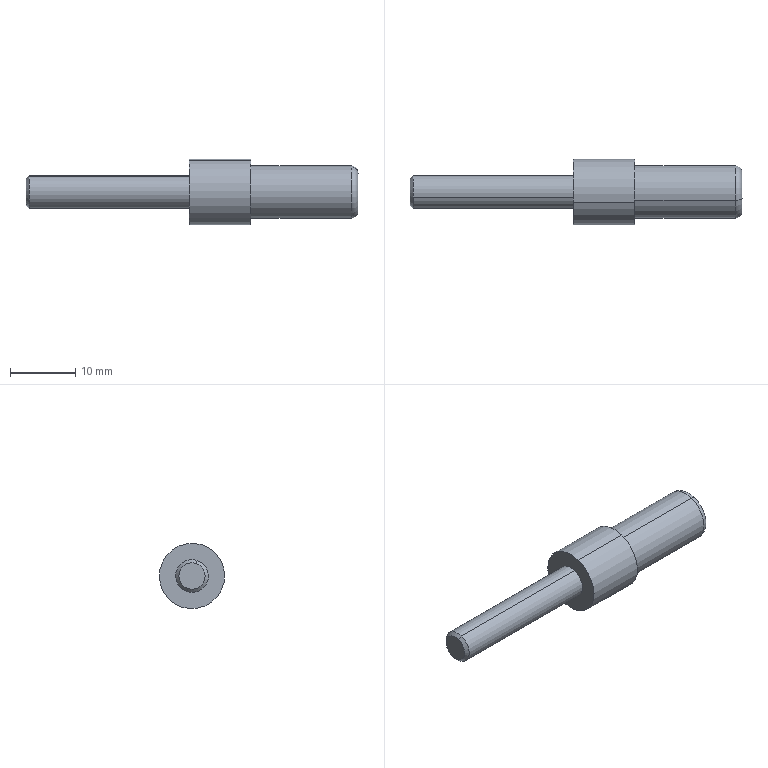Component | SolidWorks | SL010-LeftStreamline-1-1_SL010-2M-0112-000-2-1-1_SL010-CLDM5_25_B-1-1_SL010-_CLDM5_25_B_1_2-1-1 | 1 solid | 21 faces | box 50.8 x 10 x 10 mm | volume 2023 mm3 | plane 11 | cylinder 6 | torus 2 | cone 2 | commonest cylinder face diameters 8 x2 10 x2 5 x2
STEP:
#1=COLOUR_RGB('',0.7922,0.8196,0.9333);
#2=FILL_AREA_STYLE_COLOUR('',#1);
#3=FILL_AREA_STYLE('',(#2));
#4=SURFACE_STYLE_FILL_AREA(#3);
#5=SURFACE_SIDE_STYLE('',(#4));
#6=SURFACE_STYLE_USAGE(.BOTH.,#5);
#7=PRESENTATION_STYLE_ASSIGNMENT((#6));
#8=CARTESIAN_POINT('',(-5.283,-6.018,-28.334));
#9=VERTEX_POINT('',#8);
#10=CARTESIAN_POINT('',(-5.283,-5.973,-28.283));
#11=VERTEX_POINT('',#10);
#12=CARTESIAN_POINT('',(-5.283,-5.995,-28.308));
#13=DIRECTION('',(0.,0.665,0.7469));
#14=VECTOR('',#13,39.37);
#15=LINE('',#12,#14);
#16=EDGE_CURVE('',#9,#11,#15,.T.);
#17=ORIENTED_EDGE('',*,*,#16,.T.);
#18=CARTESIAN_POINT('',(-5.402,-5.973,-28.283));
#19=VERTEX_POINT('',#18);
#20=CARTESIAN_POINT('',(-5.165,-5.973,-28.283));
#21=DIRECTION('',(-1.,-0.,0.));
#22=VECTOR('',#21,39.37);
#23=LINE('',#20,#22);
#24=EDGE_CURVE('',#11,#19,#23,.T.);
#25=ORIENTED_EDGE('',*,*,#24,.T.);
#26=CARTESIAN_POINT('',(-5.402,-6.018,-28.334));
#27=VERTEX_POINT('',#26);
#28=CARTESIAN_POINT('',(-5.402,-6.018,-28.334));
#29=DIRECTION('',(0.,0.665,0.7469));
#30=VECTOR('',#29,39.37);
#31=LINE('',#28,#30);
#32=EDGE_CURVE('',#27,#19,#31,.T.);
#33=ORIENTED_EDGE('',*,*,#32,.F.);
#34=CARTESIAN_POINT('',(-5.165,-6.018,-28.334));
#35=DIRECTION('',(-1.,-0.,0.));
#36=VECTOR('',#35,39.37);
#37=LINE('',#34,#36);
#38=EDGE_CURVE('',#9,#27,#37,.T.);
#39=ORIENTED_EDGE('',*,*,#38,.F.);
#40=EDGE_LOOP('',(#17,#25,#33,#39));
#41=FACE_OUTER_BOUND('',#40,.T.);
#42=CARTESIAN_POINT('',(-5.165,-6.018,-28.334));
#43=DIRECTION('',(0.,-0.7469,0.665));
#44=DIRECTION('',(-0.,-0.665,-0.7469));
#45=AXIS2_PLACEMENT_3D('',#42,#43,#44);
#46=PLANE('',#45);
#47=ADVANCED_FACE('',(#41),#46,.T.);
#48=CARTESIAN_POINT('',(-5.283,-6.085,-28.32));
#49=VERTEX_POINT('',#48);
#50=CARTESIAN_POINT('',(-5.283,-6.051,-28.327));
#51=DIRECTION('',(-0.,0.9793,-0.2025));
#52=VECTOR('',#51,39.37);
#53=LINE('',#50,#52);
#54=EDGE_CURVE('',#49,#9,#53,.T.);
#55=ORIENTED_EDGE('',*,*,#54,.T.);
#56=ORIENTED_EDGE('',*,*,#38,.T.);
#57=CARTESIAN_POINT('',(-5.402,-6.085,-28.32));
#58=VERTEX_POINT('',#57);
#59=CARTESIAN_POINT('',(-5.402,-6.085,-28.32));
#60=DIRECTION('',(-0.,0.9793,-0.2025));
#61=VECTOR('',#60,39.37);
#62=LINE('',#59,#61);
#63=EDGE_CURVE('',#58,#27,#62,.T.);
#64=ORIENTED_EDGE('',*,*,#63,.F.);
#65=CARTESIAN_POINT('',(-5.165,-6.085,-28.32));
#66=DIRECTION('',(-1.,-0.,0.));
#67=VECTOR('',#66,39.37);
#68=LINE('',#65,#67);
#69=EDGE_CURVE('',#49,#58,#68,.T.);
#70=ORIENTED_EDGE('',*,*,#69,.F.);
#71=EDGE_LOOP('',(#55,#56,#64,#70));
#72=FACE_OUTER_BOUND('',#71,.T.);
#73=CARTESIAN_POINT('',(-5.165,-6.085,-28.32));
#74=DIRECTION('',(0.,0.2025,0.9793));
#75=DIRECTION('',(0.,-0.9793,0.2025));
#76=AXIS2_PLACEMENT_3D('',#73,#74,#75);
#77=PLANE('',#76);
#78=ADVANCED_FACE('',(#72),#77,.T.);
#79=CARTESIAN_POINT('',(-5.283,-6.106,-28.255));
#80=VERTEX_POINT('',#79);
#81=CARTESIAN_POINT('',(-5.402,-6.106,-28.255));
#82=VERTEX_POINT('',#81);
#83=CARTESIAN_POINT('',(-5.165,-6.106,-28.255));
#84=DIRECTION('',(-1.,-0.,0.));
#85=VECTOR('',#84,39.37);
#86=LINE('',#83,#85);
#87=EDGE_CURVE('',#80,#82,#86,.T.);
#88=ORIENTED_EDGE('',*,*,#87,.F.);
#89=CARTESIAN_POINT('',(-5.283,-6.096,-28.288));
#90=DIRECTION('',(-0.,0.3143,-0.9493));
#91=VECTOR('',#90,39.37);
#92=LINE('',#89,#91);
#93=EDGE_CURVE('',#80,#49,#92,.T.);
#94=ORIENTED_EDGE('',*,*,#93,.T.);
#95=ORIENTED_EDGE('',*,*,#69,.T.);
#96=CARTESIAN_POINT('',(-5.402,-6.106,-28.255));
#97=DIRECTION('',(-0.,0.3143,-0.9493));
#98=VECTOR('',#97,39.37);
#99=LINE('',#96,#98);
#100=EDGE_CURVE('',#82,#58,#99,.T.);
#101=ORIENTED_EDGE('',*,*,#100,.F.);
#102=EDGE_LOOP('',(#88,#94,#95,#101));
#103=FACE_OUTER_BOUND('',#102,.T.);
#104=CARTESIAN_POINT('',(-5.165,-6.106,-28.255));
#105=DIRECTION('',(0.,0.9493,0.3143));
#106=DIRECTION('',(0.,-0.3143,0.9493));
#107=AXIS2_PLACEMENT_3D('',#104,#105,#106);
#108=PLANE('',#107);
#109=ADVANCED_FACE('',(#103),#108,.T.);
#110=CARTESIAN_POINT('',(-5.402,-5.994,-28.218));
#111=VERTEX_POINT('',#110);
#112=CARTESIAN_POINT('',(-5.402,-5.973,-28.283));
#113=DIRECTION('',(0.,-0.3143,0.9493));
#114=VECTOR('',#113,39.37);
#115=LINE('',#112,#114);
#116=EDGE_CURVE('',#19,#111,#115,.T.);
#117=ORIENTED_EDGE('',*,*,#116,.T.);
#118=CARTESIAN_POINT('',(-5.402,-6.061,-28.204));
#119=VERTEX_POINT('',#118);
#120=CARTESIAN_POINT('',(-5.402,-5.994,-28.218));
#121=DIRECTION('',(0.,-0.9793,0.2025));
#122=VECTOR('',#121,39.37);
#123=LINE('',#120,#122);
#124=EDGE_CURVE('',#111,#119,#123,.T.);
#125=ORIENTED_EDGE('',*,*,#124,.T.);
#126=CARTESIAN_POINT('',(-5.402,-6.061,-28.204));
#127=DIRECTION('',(-0.,-0.665,-0.7469));
#128=VECTOR('',#127,39.37);
#129=LINE('',#126,#128);
#130=EDGE_CURVE('',#119,#82,#129,.T.);
#131=ORIENTED_EDGE('',*,*,#130,.T.);
#132=ORIENTED_EDGE('',*,*,#100,.T.);
#133=ORIENTED_EDGE('',*,*,#63,.T.);
#134=ORIENTED_EDGE('',*,*,#32,.T.);
#135=EDGE_LOOP('',(#117,#125,#131,#132,#133,#134));
#136=FACE_OUTER_BOUND('',#135,.T.);
#137=CARTESIAN_POINT('',(-5.402,-6.04,-28.269));
#138=DIRECTION('',(1.,0.,-0.));
#139=DIRECTION('',(0.,-0.3143,0.9493));
#140=AXIS2_PLACEMENT_3D('',#137,#138,#139);
#141=PLANE('',#140);
#142=ADVANCED_FACE('',(#136),#141,.T.);
#143=CARTESIAN_POINT('',(-5.283,-6.061,-28.204));
#144=VERTEX_POINT('',#143);
#145=CARTESIAN_POINT('',(-5.283,-6.084,-28.23));
#146=DIRECTION('',(-0.,-0.665,-0.7469));
#147=VECTOR('',#146,39.37);
#148=LINE('',#145,#147);
#149=EDGE_CURVE('',#144,#80,#148,.T.);
#150=ORIENTED_EDGE('',*,*,#149,.T.);
#151=ORIENTED_EDGE('',*,*,#87,.T.);
#152=ORIENTED_EDGE('',*,*,#130,.F.);
#153=CARTESIAN_POINT('',(-5.165,-6.061,-28.204));
#154=DIRECTION('',(-1.,-0.,0.));
#155=VECTOR('',#154,39.37);
#156=LINE('',#153,#155);
#157=EDGE_CURVE('',#144,#119,#156,.T.);
#158=ORIENTED_EDGE('',*,*,#157,.F.);
#159=EDGE_LOOP('',(#150,#151,#152,#158));
#160=FACE_OUTER_BOUND('',#159,.T.);
#161=CARTESIAN_POINT('',(-5.165,-6.061,-28.204));
#162=DIRECTION('',(-0.,0.7469,-0.665));
#163=DIRECTION('',(0.,0.665,0.7469));
#164=AXIS2_PLACEMENT_3D('',#161,#162,#163);
#165=PLANE('',#164);
#166=ADVANCED_FACE('',(#160),#165,.T.);
#167=CARTESIAN_POINT('',(-5.283,-5.994,-28.218));
#168=VERTEX_POINT('',#167);
#169=CARTESIAN_POINT('',(-5.283,-6.028,-28.211));
#170=DIRECTION('',(0.,-0.9793,0.2025));
#171=VECTOR('',#170,39.37);
#172=LINE('',#169,#171);
#173=EDGE_CURVE('',#168,#144,#172,.T.);
#174=ORIENTED_EDGE('',*,*,#173,.T.);
#175=ORIENTED_EDGE('',*,*,#157,.T.);
#176=ORIENTED_EDGE('',*,*,#124,.F.);
#177=CARTESIAN_POINT('',(-5.165,-5.994,-28.218));
#178=DIRECTION('',(-1.,-0.,0.));
#179=VECTOR('',#178,39.37);
#180=LINE('',#177,#179);
#181=EDGE_CURVE('',#168,#111,#180,.T.);
#182=ORIENTED_EDGE('',*,*,#181,.F.);
#183=EDGE_LOOP('',(#174,#175,#176,#182));
#184=FACE_OUTER_BOUND('',#183,.T.);
#185=CARTESIAN_POINT('',(-5.165,-5.994,-28.218));
#186=DIRECTION('',(-0.,-0.2025,-0.9793));
#187=DIRECTION('',(-0.,0.9793,-0.2025));
#188=AXIS2_PLACEMENT_3D('',#185,#186,#187);
#189=PLANE('',#188);
#190=ADVANCED_FACE('',(#184),#189,.T.);
#191=CARTESIAN_POINT('',(-5.283,-5.983,-28.251));
#192=DIRECTION('',(0.,-0.3143,0.9493));
#193=VECTOR('',#192,39.37);
#194=LINE('',#191,#193);
#195=EDGE_CURVE('',#11,#168,#194,.T.);
#196=ORIENTED_EDGE('',*,*,#195,.T.);
#197=ORIENTED_EDGE('',*,*,#181,.T.);
#198=ORIENTED_EDGE('',*,*,#116,.F.);
#199=ORIENTED_EDGE('',*,*,#24,.F.);
#200=EDGE_LOOP('',(#196,#197,#198,#199));
#201=FACE_OUTER_BOUND('',#200,.T.);
#202=CARTESIAN_POINT('',(-5.165,-5.973,-28.283));
#203=DIRECTION('',(0.,-0.9493,-0.3143));
#204=DIRECTION('',(-0.,0.3143,-0.9493));
#205=AXIS2_PLACEMENT_3D('',#202,#203,#204);
#206=PLANE('',#205);
#207=ADVANCED_FACE('',(#201),#206,.T.);
#208=CARTESIAN_POINT('',(-5.283,-6.002,-28.381));
#209=VERTEX_POINT('',#208);
#210=CARTESIAN_POINT('',(-5.283,-6.077,-28.157));
#211=VERTEX_POINT('',#210);
#212=CARTESIAN_POINT('',(-5.283,-6.04,-28.269));
#213=DIRECTION('',(-1.,-0.,0.));
#214=DIRECTION('',(0.,0.3143,-0.9493));
#215=AXIS2_PLACEMENT_3D('',#212,#213,#214);
#216=CIRCLE('',#215,0.1181);
#217=EDGE_CURVE('',#209,#211,#216,.T.);
#218=ORIENTED_EDGE('',*,*,#217,.F.);
#219=CARTESIAN_POINT('',(-5.283,-6.04,-28.269));
#220=DIRECTION('',(-1.,-0.,0.));
#221=DIRECTION('',(0.,0.3143,-0.9493));
#222=AXIS2_PLACEMENT_3D('',#219,#220,#221);
#223=CIRCLE('',#222,0.1181);
#224=EDGE_CURVE('',#211,#209,#223,.T.);
#225=ORIENTED_EDGE('',*,*,#224,.F.);
#226=EDGE_LOOP('',(#218,#225));
#227=FACE_OUTER_BOUND('',#226,.T.);
#228=ORIENTED_EDGE('',*,*,#195,.F.);
#229=ORIENTED_EDGE('',*,*,#16,.F.);
#230=ORIENTED_EDGE('',*,*,#54,.F.);
#231=ORIENTED_EDGE('',*,*,#93,.F.);
#232=ORIENTED_EDGE('',*,*,#149,.F.);
#233=ORIENTED_EDGE('',*,*,#173,.F.);
#234=EDGE_LOOP('',(#228,#229,#230,#231,#232,#233));
#235=FACE_BOUND('',#234,.T.);
#236=CARTESIAN_POINT('',(-5.283,-6.04,-28.269));
#237=DIRECTION('',(-1.,-0.,0.));
#238=DIRECTION('',(-0.,0.3143,-0.9493));
#239=AXIS2_PLACEMENT_3D('',#236,#237,#238);
#240=PLANE('',#239);
#241=ADVANCED_FACE('',(#227,#235),#240,.F.);
#242=ORIENTED_EDGE('',*,*,#224,.T.);
#243=CARTESIAN_POINT('',(-5.323,-5.99,-28.419));
#244=VERTEX_POINT('',#243);
#245=CARTESIAN_POINT('',(-5.283,-6.002,-28.381));
#246=CARTESIAN_POINT('',(-5.283,-5.999,-28.391));
#247=CARTESIAN_POINT('',(-5.288,-5.996,-28.401));
#248=CARTESIAN_POINT('',(-5.302,-5.991,-28.415));
#249=CARTESIAN_POINT('',(-5.313,-5.99,-28.419));
#250=CARTESIAN_POINT('',(-5.323,-5.99,-28.419));
#251=B_SPLINE_CURVE_WITH_KNOTS('',3,(#245,#246,#247,#248,#249,#250),.UNSPECIFIED.,.F.,.F.,(4,2,4),(0.,0.7854,1.571),.UNSPECIFIED.);
#252=EDGE_CURVE('',#209,#244,#251,.T.);
#253=ORIENTED_EDGE('',*,*,#252,.T.);
#254=CARTESIAN_POINT('',(-5.323,-6.089,-28.12));
#255=VERTEX_POINT('',#254);
#256=CARTESIAN_POINT('',(-5.323,-6.04,-28.269));
#257=DIRECTION('',(-1.,-0.,0.));
#258=DIRECTION('',(0.,0.3143,-0.9493));
#259=AXIS2_PLACEMENT_3D('',#256,#257,#258);
#260=CIRCLE('',#259,0.1575);
#261=EDGE_CURVE('',#255,#244,#260,.T.);
#262=ORIENTED_EDGE('',*,*,#261,.F.);
#263=CARTESIAN_POINT('',(-5.283,-6.077,-28.157));
#264=CARTESIAN_POINT('',(-5.283,-6.08,-28.147));
#265=CARTESIAN_POINT('',(-5.288,-6.083,-28.137));
#266=CARTESIAN_POINT('',(-5.302,-6.088,-28.124));
#267=CARTESIAN_POINT('',(-5.313,-6.089,-28.12));
#268=CARTESIAN_POINT('',(-5.323,-6.089,-28.12));
#269=B_SPLINE_CURVE_WITH_KNOTS('',3,(#263,#264,#265,#266,#267,#268),.UNSPECIFIED.,.F.,.F.,(4,2,4),(0.,0.7854,1.571),.UNSPECIFIED.);
#270=EDGE_CURVE('',#211,#255,#269,.T.);
#271=ORIENTED_EDGE('',*,*,#270,.F.);
#272=EDGE_LOOP('',(#242,#253,#262,#271));
#273=FACE_OUTER_BOUND('',#272,.T.);
#274=CARTESIAN_POINT('',(-5.323,-6.04,-28.269));
#275=DIRECTION('',(-1.,-0.,0.));
#276=DIRECTION('',(0.,-0.9493,-0.3143));
#277=AXIS2_PLACEMENT_3D('',#274,#275,#276);
#278=TOROIDAL_SURFACE('',#277,0.1181,0.03937);
#279=ADVANCED_FACE('',(#273),#278,.T.);
#280=CARTESIAN_POINT('',(-5.323,-6.04,-28.269));
#281=DIRECTION('',(-1.,-0.,0.));
#282=DIRECTION('',(0.,0.3143,-0.9493));
#283=AXIS2_PLACEMENT_3D('',#280,#281,#282);
#284=CIRCLE('',#283,0.1575);
#285=EDGE_CURVE('',#244,#255,#284,.T.);
#286=ORIENTED_EDGE('',*,*,#285,.F.);
#287=ORIENTED_EDGE('',*,*,#252,.F.);
#288=ORIENTED_EDGE('',*,*,#217,.T.);
#289=ORIENTED_EDGE('',*,*,#270,.T.);
#290=EDGE_LOOP('',(#286,#287,#288,#289));
#291=FACE_OUTER_BOUND('',#290,.T.);
#292=CARTESIAN_POINT('',(-5.323,-6.04,-28.269));
#293=DIRECTION('',(-1.,-0.,0.));
#294=DIRECTION('',(-0.,0.9493,0.3143));
#295=AXIS2_PLACEMENT_3D('',#292,#293,#294);
#296=TOROIDAL_SURFACE('',#295,0.1181,0.03937);
#297=ADVANCED_FACE('',(#291),#296,.T.);
#298=CARTESIAN_POINT('',(-5.929,-5.99,-28.419));
#299=VERTEX_POINT('',#298);
#300=CARTESIAN_POINT('',(-5.929,-6.089,-28.12));
#301=VERTEX_POINT('',#300);
#302=CARTESIAN_POINT('',(-5.929,-6.04,-28.269));
#303=DIRECTION('',(-1.,-0.,0.));
#304=DIRECTION('',(0.,0.3143,-0.9493));
#305=AXIS2_PLACEMENT_3D('',#302,#303,#304);
#306=CIRCLE('',#305,0.1575);
#307=EDGE_CURVE('',#299,#301,#306,.T.);
#308=ORIENTED_EDGE('',*,*,#307,.F.);
#309=CARTESIAN_POINT('',(-5.929,-5.99,-28.419));
#310=DIRECTION('',(1.,0.,-0.));
#311=VECTOR('',#310,39.37);
#312=LINE('',#309,#311);
#313=EDGE_CURVE('',#299,#244,#312,.T.);
#314=ORIENTED_EDGE('',*,*,#313,.T.);
#315=ORIENTED_EDGE('',*,*,#285,.T.);
#316=CARTESIAN_POINT('',(-5.929,-6.089,-28.12));
#317=DIRECTION('',(1.,0.,-0.));
#318=VECTOR('',#317,39.37);
#319=LINE('',#316,#318);
#320=EDGE_CURVE('',#301,#255,#319,.T.);
#321=ORIENTED_EDGE('',*,*,#320,.F.);
#322=EDGE_LOOP('',(#308,#314,#315,#321));
#323=FACE_OUTER_BOUND('',#322,.T.);
#324=CARTESIAN_POINT('',(-7.283,-6.04,-28.269));
#325=DIRECTION('',(1.,0.,-0.));
#326=DIRECTION('',(0.,0.9493,0.3143));
#327=AXIS2_PLACEMENT_3D('',#324,#325,#326);
#328=CYLINDRICAL_SURFACE('',#327,0.1575);
#329=ADVANCED_FACE('',(#323),#328,.T.);
#330=ORIENTED_EDGE('',*,*,#261,.T.);
#331=ORIENTED_EDGE('',*,*,#313,.F.);
#332=CARTESIAN_POINT('',(-5.929,-6.04,-28.269));
#333=DIRECTION('',(-1.,-0.,0.));
#334=DIRECTION('',(0.,0.3143,-0.9493));
#335=AXIS2_PLACEMENT_3D('',#332,#333,#334);
#336=CIRCLE('',#335,0.1575);
#337=EDGE_CURVE('',#301,#299,#336,.T.);
#338=ORIENTED_EDGE('',*,*,#337,.F.);
#339=ORIENTED_EDGE('',*,*,#320,.T.);
#340=EDGE_LOOP('',(#330,#331,#338,#339));
#341=FACE_OUTER_BOUND('',#340,.T.);
#342=CARTESIAN_POINT('',(-7.283,-6.04,-28.269));
#343=DIRECTION('',(1.,0.,-0.));
#344=DIRECTION('',(0.,-0.9493,-0.3143));
#345=AXIS2_PLACEMENT_3D('',#342,#343,#344);
#346=CYLINDRICAL_SURFACE('',#345,0.1575);
#347=ADVANCED_FACE('',(#341),#346,.T.);
#348=CARTESIAN_POINT('',(-5.929,-5.978,-28.456));
#349=VERTEX_POINT('',#348);
#350=CARTESIAN_POINT('',(-5.929,-6.101,-28.082));
#351=VERTEX_POINT('',#350);
#352=CARTESIAN_POINT('',(-5.929,-6.04,-28.269));
#353=DIRECTION('',(-1.,-0.,0.));
#354=DIRECTION('',(0.,0.3143,-0.9493));
#355=AXIS2_PLACEMENT_3D('',#352,#353,#354);
#356=CIRCLE('',#355,0.1969);
#357=EDGE_CURVE('',#349,#351,#356,.T.);
#358=ORIENTED_EDGE('',*,*,#357,.F.);
#359=CARTESIAN_POINT('',(-5.929,-6.04,-28.269));
#360=DIRECTION('',(-1.,-0.,0.));
#361=DIRECTION('',(0.,0.3143,-0.9493));
#362=AXIS2_PLACEMENT_3D('',#359,#360,#361);
#363=CIRCLE('',#362,0.1969);
#364=EDGE_CURVE('',#351,#349,#363,.T.);
#365=ORIENTED_EDGE('',*,*,#364,.F.);
#366=EDGE_LOOP('',(#358,#365));
#367=FACE_OUTER_BOUND('',#366,.T.);
#368=ORIENTED_EDGE('',*,*,#307,.T.);
#369=ORIENTED_EDGE('',*,*,#337,.T.);
#370=EDGE_LOOP('',(#368,#369));
#371=FACE_BOUND('',#370,.T.);
#372=CARTESIAN_POINT('',(-5.929,-6.189,-28.319));
#373=DIRECTION('',(-1.,-0.,0.));
#374=DIRECTION('',(-0.,0.3143,-0.9493));
#375=AXIS2_PLACEMENT_3D('',#372,#373,#374);
#376=PLANE('',#375);
#377=ADVANCED_FACE('',(#367,#371),#376,.F.);
#378=ORIENTED_EDGE('',*,*,#364,.T.);
#379=CARTESIAN_POINT('',(-6.299,-5.978,-28.456));
#380=VERTEX_POINT('',#379);
#381=CARTESIAN_POINT('',(-6.299,-5.978,-28.456));
#382=DIRECTION('',(1.,0.,-0.));
#383=VECTOR('',#382,39.37);
#384=LINE('',#381,#383);
#385=EDGE_CURVE('',#380,#349,#384,.T.);
#386=ORIENTED_EDGE('',*,*,#385,.F.);
#387=CARTESIAN_POINT('',(-6.299,-6.101,-28.082));
#388=VERTEX_POINT('',#387);
#389=CARTESIAN_POINT('',(-6.299,-6.04,-28.269));
#390=DIRECTION('',(-1.,-0.,0.));
#391=DIRECTION('',(0.,0.3143,-0.9493));
#392=AXIS2_PLACEMENT_3D('',#389,#390,#391);
#393=CIRCLE('',#392,0.1969);
#394=EDGE_CURVE('',#388,#380,#393,.T.);
#395=ORIENTED_EDGE('',*,*,#394,.F.);
#396=CARTESIAN_POINT('',(-6.299,-6.101,-28.082));
#397=DIRECTION('',(1.,0.,-0.));
#398=VECTOR('',#397,39.37);
#399=LINE('',#396,#398);
#400=EDGE_CURVE('',#388,#351,#399,.T.);
#401=ORIENTED_EDGE('',*,*,#400,.T.);
#402=EDGE_LOOP('',(#378,#386,#395,#401));
#403=FACE_OUTER_BOUND('',#402,.T.);
#404=CARTESIAN_POINT('',(-7.283,-6.04,-28.269));
#405=DIRECTION('',(1.,0.,-0.));
#406=DIRECTION('',(0.,-0.9493,-0.3143));
#407=AXIS2_PLACEMENT_3D('',#404,#405,#406);
#408=CYLINDRICAL_SURFACE('',#407,0.1969);
#409=ADVANCED_FACE('',(#403),#408,.T.);
#410=CARTESIAN_POINT('',(-6.299,-6.04,-28.269));
#411=DIRECTION('',(-1.,-0.,0.));
#412=DIRECTION('',(0.,0.3143,-0.9493));
#413=AXIS2_PLACEMENT_3D('',#410,#411,#412);
#414=CIRCLE('',#413,0.1969);
#415=EDGE_CURVE('',#380,#388,#414,.T.);
#416=ORIENTED_EDGE('',*,*,#415,.F.);
#417=ORIENTED_EDGE('',*,*,#385,.T.);
#418=ORIENTED_EDGE('',*,*,#357,.T.);
#419=ORIENTED_EDGE('',*,*,#400,.F.);
#420=EDGE_LOOP('',(#416,#417,#418,#419));
#421=FACE_OUTER_BOUND('',#420,.T.);
#422=CARTESIAN_POINT('',(-7.283,-6.04,-28.269));
#423=DIRECTION('',(1.,0.,-0.));
#424=DIRECTION('',(0.,0.9493,0.3143));
#425=AXIS2_PLACEMENT_3D('',#422,#423,#424);
#426=CYLINDRICAL_SURFACE('',#425,0.1969);
#427=ADVANCED_FACE('',(#421),#426,.T.);
#428=CARTESIAN_POINT('',(-6.299,-6.009,-28.363));
#429=VERTEX_POINT('',#428);
#430=CARTESIAN_POINT('',(-6.299,-6.07,-28.176));
#431=VERTEX_POINT('',#430);
#432=CARTESIAN_POINT('',(-6.299,-6.04,-28.269));
#433=DIRECTION('',(-1.,-0.,0.));
#434=DIRECTION('',(0.,0.3143,-0.9493));
#435=AXIS2_PLACEMENT_3D('',#432,#433,#434);
#436=CIRCLE('',#435,0.09843);
#437=EDGE_CURVE('',#429,#431,#436,.T.);
#438=ORIENTED_EDGE('',*,*,#437,.F.);
#439=CARTESIAN_POINT('',(-6.299,-6.04,-28.269));
#440=DIRECTION('',(-1.,-0.,0.));
#441=DIRECTION('',(0.,0.3143,-0.9493));
#442=AXIS2_PLACEMENT_3D('',#439,#440,#441);
#443=CIRCLE('',#442,0.09843);
#444=EDGE_CURVE('',#431,#429,#443,.T.);
#445=ORIENTED_EDGE('',*,*,#444,.F.);
#446=EDGE_LOOP('',(#438,#445));
#447=FACE_BOUND('',#446,.T.);
#448=ORIENTED_EDGE('',*,*,#415,.T.);
#449=ORIENTED_EDGE('',*,*,#394,.T.);
#450=EDGE_LOOP('',(#448,#449));
#451=FACE_OUTER_BOUND('',#450,.T.);
#452=CARTESIAN_POINT('',(-6.299,-6.226,-28.331));
#453=DIRECTION('',(1.,0.,-0.));
#454=DIRECTION('',(0.,-0.3143,0.9493));
#455=AXIS2_PLACEMENT_3D('',#452,#453,#454);
#456=PLANE('',#455);
#457=ADVANCED_FACE('',(#447,#451),#456,.F.);
#458=ORIENTED_EDGE('',*,*,#444,.T.);
#459=CARTESIAN_POINT('',(-7.264,-6.009,-28.363));
#460=VERTEX_POINT('',#459);
#461=CARTESIAN_POINT('',(-7.264,-6.009,-28.363));
#462=DIRECTION('',(1.,0.,-0.));
#463=VECTOR('',#462,39.37);
#464=LINE('',#461,#463);
#465=EDGE_CURVE('',#460,#429,#464,.T.);
#466=ORIENTED_EDGE('',*,*,#465,.F.);
#467=CARTESIAN_POINT('',(-7.264,-6.07,-28.176));
#468=VERTEX_POINT('',#467);
#469=CARTESIAN_POINT('',(-7.264,-6.04,-28.269));
#470=DIRECTION('',(-1.,-0.,0.));
#471=DIRECTION('',(0.,0.3143,-0.9493));
#472=AXIS2_PLACEMENT_3D('',#469,#470,#471);
#473=CIRCLE('',#472,0.09843);
#474=EDGE_CURVE('',#468,#460,#473,.T.);
#475=ORIENTED_EDGE('',*,*,#474,.F.);
#476=CARTESIAN_POINT('',(-7.264,-6.07,-28.176));
#477=DIRECTION('',(1.,0.,-0.));
#478=VECTOR('',#477,39.37);
#479=LINE('',#476,#478);
#480=EDGE_CURVE('',#468,#431,#479,.T.);
#481=ORIENTED_EDGE('',*,*,#480,.T.);
#482=EDGE_LOOP('',(#458,#466,#475,#481));
#483=FACE_OUTER_BOUND('',#482,.T.);
#484=CARTESIAN_POINT('',(-7.283,-6.04,-28.269));
#485=DIRECTION('',(1.,0.,-0.));
#486=DIRECTION('',(0.,-0.9493,-0.3143));
#487=AXIS2_PLACEMENT_3D('',#484,#485,#486);
#488=CYLINDRICAL_SURFACE('',#487,0.09843);
#489=ADVANCED_FACE('',(#483),#488,.T.);
#490=CARTESIAN_POINT('',(-7.264,-6.04,-28.269));
#491=DIRECTION('',(-1.,-0.,0.));
#492=DIRECTION('',(0.,0.3143,-0.9493));
#493=AXIS2_PLACEMENT_3D('',#490,#491,#492);
#494=CIRCLE('',#493,0.09843);
#495=EDGE_CURVE('',#460,#468,#494,.T.);
#496=ORIENTED_EDGE('',*,*,#495,.F.);
#497=ORIENTED_EDGE('',*,*,#465,.T.);
#498=ORIENTED_EDGE('',*,*,#437,.T.);
#499=ORIENTED_EDGE('',*,*,#480,.F.);
#500=EDGE_LOOP('',(#496,#497,#498,#499));
#501=FACE_OUTER_BOUND('',#500,.T.);
#502=CARTESIAN_POINT('',(-7.283,-6.04,-28.269));
#503=DIRECTION('',(1.,0.,-0.));
#504=DIRECTION('',(0.,0.9493,0.3143));
#505=AXIS2_PLACEMENT_3D('',#502,#503,#504);
#506=CYLINDRICAL_SURFACE('',#505,0.09843);
#507=ADVANCED_FACE('',(#501),#506,.T.);
#508=CARTESIAN_POINT('',(-7.283,-6.015,-28.344));
#509=VERTEX_POINT('',#508);
#510=CARTESIAN_POINT('',(-7.283,-6.064,-28.194));
#511=VERTEX_POINT('',#510);
#512=CARTESIAN_POINT('',(-7.283,-6.04,-28.269));
#513=DIRECTION('',(-1.,-0.,0.));
#514=DIRECTION('',(0.,0.3143,-0.9493));
#515=AXIS2_PLACEMENT_3D('',#512,#513,#514);
#516=CIRCLE('',#515,0.07911);
#517=EDGE_CURVE('',#509,#511,#516,.T.);
#518=ORIENTED_EDGE('',*,*,#517,.F.);
#519=CARTESIAN_POINT('',(-7.283,-6.015,-28.344));
#520=DIRECTION('',(0.7071,0.2223,-0.6713));
#521=VECTOR('',#520,39.37);
#522=LINE('',#519,#521);
#523=EDGE_CURVE('',#509,#460,#522,.T.);
#524=ORIENTED_EDGE('',*,*,#523,.T.);
#525=ORIENTED_EDGE('',*,*,#495,.T.);
#526=CARTESIAN_POINT('',(-7.283,-6.064,-28.194));
#527=DIRECTION('',(0.7071,-0.2223,0.6713));
#528=VECTOR('',#527,39.37);
#529=LINE('',#526,#528);
#530=EDGE_CURVE('',#511,#468,#529,.T.);
#531=ORIENTED_EDGE('',*,*,#530,.F.);
#532=EDGE_LOOP('',(#518,#524,#525,#531));
#533=FACE_OUTER_BOUND('',#532,.T.);
#534=CARTESIAN_POINT('',(-7.264,-6.04,-28.269));
#535=DIRECTION('',(1.,0.,-0.));
#536=DIRECTION('',(0.,0.9493,0.3143));
#537=AXIS2_PLACEMENT_3D('',#534,#535,#536);
#538=CONICAL_SURFACE('',#537,0.09843,0.7854);
#539=ADVANCED_FACE('',(#533),#538,.T.);
#540=ORIENTED_EDGE('',*,*,#474,.T.);
#541=ORIENTED_EDGE('',*,*,#523,.F.);
#542=CARTESIAN_POINT('',(-7.283,-6.04,-28.269));
#543=DIRECTION('',(-1.,-0.,0.));
#544=DIRECTION('',(0.,0.3143,-0.9493));
#545=AXIS2_PLACEMENT_3D('',#542,#543,#544);
#546=CIRCLE('',#545,0.07911);
#547=EDGE_CURVE('',#511,#509,#546,.T.);
#548=ORIENTED_EDGE('',*,*,#547,.F.);
#549=ORIENTED_EDGE('',*,*,#530,.T.);
#550=EDGE_LOOP('',(#540,#541,#548,#549));
#551=FACE_OUTER_BOUND('',#550,.T.);
#552=CARTESIAN_POINT('',(-7.264,-6.04,-28.269));
#553=DIRECTION('',(1.,0.,-0.));
#554=DIRECTION('',(0.,-0.9493,-0.3143));
#555=AXIS2_PLACEMENT_3D('',#552,#553,#554);
#556=CONICAL_SURFACE('',#555,0.09843,0.7854);
#557=ADVANCED_FACE('',(#551),#556,.T.);
#558=ORIENTED_EDGE('',*,*,#517,.T.);
#559=ORIENTED_EDGE('',*,*,#547,.T.);
#560=EDGE_LOOP('',(#558,#559));
#561=FACE_OUTER_BOUND('',#560,.T.);
#562=CARTESIAN_POINT('',(-7.283,-6.115,-28.294));
#563=DIRECTION('',(1.,0.,-0.));
#564=DIRECTION('',(0.,-0.3143,0.9493));
#565=AXIS2_PLACEMENT_3D('',#562,#563,#564);
#566=PLANE('',#565);
#567=ADVANCED_FACE('',(#561),#566,.F.);
#568=CLOSED_SHELL('',(#47,#78,#109,#142,#166,#190,#207,#241,#279,#297,#329,#347,#377,#409,#427,#457,#489,#507,#539,#557,#567));
#569=MANIFOLD_SOLID_BREP('',#568);
#570=STYLED_ITEM('',(#7),#569);
#571=PRESENTATION_LAYER_ASSIGNMENT('','',(#570));
#572=(LENGTH_UNIT()NAMED_UNIT(*)SI_UNIT($,.METRE.));
#573=LENGTH_MEASURE_WITH_UNIT(LENGTH_MEASURE(0.0254),#572);
#574=DIMENSIONAL_EXPONENTS(1.,0.,0.,0.,0.,0.,0.);
#575=(CONVERSION_BASED_UNIT('',#573)LENGTH_UNIT()NAMED_UNIT(#574));
#576=UNCERTAINTY_MEASURE_WITH_UNIT(LENGTH_MEASURE(0.00001),#575,'','');
#577=(NAMED_UNIT(*)PLANE_ANGLE_UNIT()SI_UNIT($,.RADIAN.));
#578=(NAMED_UNIT(*)SI_UNIT($,.STERADIAN.)SOLID_ANGLE_UNIT());
#579=(GEOMETRIC_REPRESENTATION_CONTEXT(3)GLOBAL_UNCERTAINTY_ASSIGNED_CONTEXT((#576))GLOBAL_UNIT_ASSIGNED_CONTEXT((#575,#577,#578))REPRESENTATION_CONTEXT('',''));
#580=MECHANICAL_DESIGN_GEOMETRIC_PRESENTATION_REPRESENTATION('',(#570),#579);
#581=CARTESIAN_POINT('',(0.,0.,0.));
#582=DIRECTION('',(0.,0.,1.));
#583=DIRECTION('',(1.,0.,0.));
#584=AXIS2_PLACEMENT_3D('',#581,#582,#583);
#585=(LENGTH_UNIT()NAMED_UNIT(*)SI_UNIT($,.METRE.));
#586=LENGTH_MEASURE_WITH_UNIT(LENGTH_MEASURE(0.0254),#585);
#587=DIMENSIONAL_EXPONENTS(1.,0.,0.,0.,0.,0.,0.);
#588=(CONVERSION_BASED_UNIT('',#586)LENGTH_UNIT()NAMED_UNIT(#587));
#589=UNCERTAINTY_MEASURE_WITH_UNIT(LENGTH_MEASURE(0.00001),#588,'','');
#590=(NAMED_UNIT(*)PLANE_ANGLE_UNIT()SI_UNIT($,.RADIAN.));
#591=(NAMED_UNIT(*)SI_UNIT($,.STERADIAN.)SOLID_ANGLE_UNIT());
#592=(GEOMETRIC_REPRESENTATION_CONTEXT(3)GLOBAL_UNCERTAINTY_ASSIGNED_CONTEXT((#589))GLOBAL_UNIT_ASSIGNED_CONTEXT((#588,#590,#591))REPRESENTATION_CONTEXT('',''));
#593=ADVANCED_BREP_SHAPE_REPRESENTATION('',(#569,#584),#592);